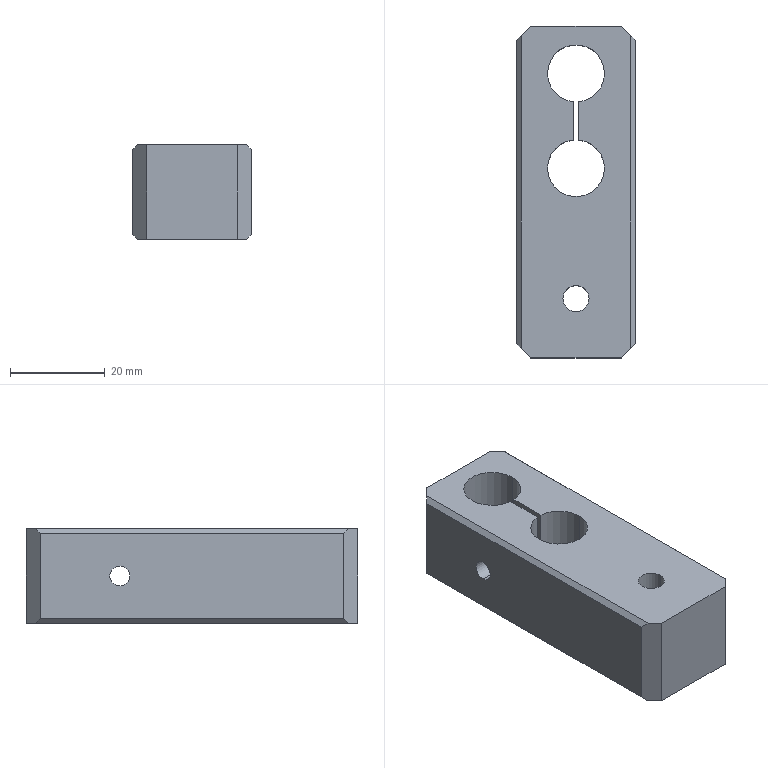Component | SolidWorks | 56-1 | 1 solid | 31 faces | box 25 x 70 x 20 mm | volume 28604 mm3 | plane 17 | cylinder 14 | commonest cylinder face diameters 12 x6 5.5 x4 4.2 x2 10 x2
build123d program:
from build123d import *

# Parameters (mm, degrees)
SKETCH1_W                                            = 25
SKETCH1_H                                            = 70
SKETCH1_R                                            = 6
BOSS_EXTRUDE1_DEPTH                                  = 20
CHAMFER1_SIZE                                        = 3
SKETCH2_W                                            = 1
SKETCH2_H                                            = 16.444
CUT_EXTRUDE1_DEPTH                                   = 20
M5_HEX_SOCKET_HEAD_CAP_SCREW_COUNTERBORE_D           = 5.5
M5_HEX_SOCKET_HEAD_CAP_SCREW_COUNTERBORE_DEPTH       = 12
M5_HEX_SOCKET_HEAD_CAP_SCREW_COUNTERBORE_CBORE_D     = 10
M5_HEX_SOCKET_HEAD_CAP_SCREW_COUNTERBORE_CBORE_DEPTH = 5.4
M5_TAPPED_HOLE1_D                                    = 4.2
M5_TAPPED_HOLE1_DEPTH                                = 14
M5_TAPPED_HOLE1_TIP                                  = 1.262
SKETCH6_R                                            = 2.75
CUT_EXTRUDE2_DEPTH                                   = 20
CHAMFER2_SIZE                                        = 3
CHAMFER3_SIZE                                        = 1


with BuildPart() as part:
    # Sketch1 → Boss-Extrude1 (new body)
    with BuildSketch(Plane.XY):
        with Locations((0, -5)):
            Rectangle(SKETCH1_W, SKETCH1_H)
        Circle(SKETCH1_R, mode=Mode.SUBTRACT)
        with Locations((0, 20)):
            Circle(SKETCH1_R, mode=Mode.SUBTRACT)
    extrude(amount=BOSS_EXTRUDE1_DEPTH)

    # Chamfer1
    chamfer1_edges = [part.edges().sort_by_distance(p)[0] for p in [
        (-12.5, 30, 10),
        (12.5, 30, 10),
    ]]
    chamfer(chamfer1_edges, length=CHAMFER1_SIZE)

    # Sketch2 → Cut-Extrude1 (cut)
    with BuildSketch(Plane.XY.offset(20)):
        with Locations((0, 8.896)):
            Rectangle(SKETCH2_W, SKETCH2_H)
    extrude(amount=-CUT_EXTRUDE1_DEPTH, mode=Mode.SUBTRACT)

    # M5 Hex Socket Head Cap Screw Counterbore
    with Locations(Plane(origin=(12.5, 10.226, 10), x_dir=(0, 1, 0), z_dir=(1, 0, 0))):
        with Locations((0, 0)):
            CounterBoreHole(M5_HEX_SOCKET_HEAD_CAP_SCREW_COUNTERBORE_D / 2, M5_HEX_SOCKET_HEAD_CAP_SCREW_COUNTERBORE_CBORE_D / 2, M5_HEX_SOCKET_HEAD_CAP_SCREW_COUNTERBORE_CBORE_DEPTH, depth=M5_HEX_SOCKET_HEAD_CAP_SCREW_COUNTERBORE_DEPTH)

    # M5 Tapped Hole1
    with Locations(Plane(origin=(-0.5, 0, 0), x_dir=(0, 0, -1), z_dir=(1, 0, 0))):
        with Locations((-10, 10.226)):
            Hole(M5_TAPPED_HOLE1_D / 2, depth=M5_TAPPED_HOLE1_DEPTH)
            with Locations((0, 0, -(M5_TAPPED_HOLE1_DEPTH + M5_TAPPED_HOLE1_TIP / 2))):  # 118° drill point
                Cone(0, M5_TAPPED_HOLE1_D / 2, M5_TAPPED_HOLE1_TIP, mode=Mode.SUBTRACT)

    # Sketch6 → Cut-Extrude2 (cut)
    with BuildSketch(Plane.XY.offset(20)):
        with Locations((0, -27.5)):
            Circle(SKETCH6_R)
    extrude(amount=-CUT_EXTRUDE2_DEPTH, mode=Mode.SUBTRACT)

    # Chamfer2
    chamfer2_edges = [part.edges().sort_by_distance(p)[0] for p in [
        (12.5, -40, 10),
        (-12.5, -40, 10),
    ]]
    chamfer(chamfer2_edges, length=CHAMFER2_SIZE)

    # Chamfer3
    chamfer3_edges = [part.edges().sort_by_distance(p)[0] for p in [
        (-12.5, -5, 0),
        (-12.5, -5, 20),
        (12.5, -5, 0),
        (12.5, -5, 20),
    ]]
    chamfer(chamfer3_edges, length=CHAMFER3_SIZE)


solid = part.part

# Placed as in the assembly
solid = solid.moved(Location((0, -38, 253.966), (0, 0, 0)))
STEP:
#1=COLOUR_RGB('',0.7922,0.8196,0.9333);
#2=FILL_AREA_STYLE_COLOUR('',#1);
#3=FILL_AREA_STYLE('',(#2));
#4=SURFACE_STYLE_FILL_AREA(#3);
#5=SURFACE_SIDE_STYLE('',(#4));
#6=SURFACE_STYLE_USAGE(.BOTH.,#5);
#7=PRESENTATION_STYLE_ASSIGNMENT((#6));
#8=CARTESIAN_POINT('',(-0.1083,-2.579,9.999));
#9=VERTEX_POINT('',#8);
#10=CARTESIAN_POINT('',(0.1083,-2.579,9.999));
#11=VERTEX_POINT('',#10);
#12=CARTESIAN_POINT('',(0.,-2.579,9.999));
#13=DIRECTION('',(0.,0.,1.));
#14=DIRECTION('',(1.,0.,0.));
#15=AXIS2_PLACEMENT_3D('',#12,#13,#14);
#16=CIRCLE('',#15,0.1083);
#17=EDGE_CURVE('',#9,#11,#16,.T.);
#18=ORIENTED_EDGE('',*,*,#17,.F.);
#19=CARTESIAN_POINT('',(-0.1083,-2.579,10.786));
#20=VERTEX_POINT('',#19);
#21=CARTESIAN_POINT('',(-0.1083,-2.579,9.999));
#22=DIRECTION('',(0.,0.,1.));
#23=VECTOR('',#22,39.37);
#24=LINE('',#21,#23);
#25=EDGE_CURVE('',#9,#20,#24,.T.);
#26=ORIENTED_EDGE('',*,*,#25,.T.);
#27=CARTESIAN_POINT('',(0.1083,-2.579,10.786));
#28=VERTEX_POINT('',#27);
#29=CARTESIAN_POINT('',(0.,-2.579,10.786));
#30=DIRECTION('',(0.,0.,1.));
#31=DIRECTION('',(1.,0.,0.));
#32=AXIS2_PLACEMENT_3D('',#29,#30,#31);
#33=CIRCLE('',#32,0.1083);
#34=EDGE_CURVE('',#20,#28,#33,.T.);
#35=ORIENTED_EDGE('',*,*,#34,.T.);
#36=CARTESIAN_POINT('',(0.1083,-2.579,9.999));
#37=DIRECTION('',(0.,0.,1.));
#38=VECTOR('',#37,39.37);
#39=LINE('',#36,#38);
#40=EDGE_CURVE('',#11,#28,#39,.T.);
#41=ORIENTED_EDGE('',*,*,#40,.F.);
#42=EDGE_LOOP('',(#18,#26,#35,#41));
#43=FACE_OUTER_BOUND('',#42,.T.);
#44=CARTESIAN_POINT('',(0.,-2.579,9.999));
#45=DIRECTION('',(0.,0.,1.));
#46=DIRECTION('',(1.,0.,0.));
#47=AXIS2_PLACEMENT_3D('',#44,#45,#46);
#48=CYLINDRICAL_SURFACE('',#47,0.1083);
#49=ADVANCED_FACE('',(#43),#48,.F.);
#50=CARTESIAN_POINT('',(-0.4921,-1.093,10.475));
#51=VERTEX_POINT('',#50);
#52=CARTESIAN_POINT('',(-0.4921,-1.093,10.31));
#53=VERTEX_POINT('',#52);
#54=CARTESIAN_POINT('',(-0.4921,-1.093,10.392));
#55=DIRECTION('',(1.,0.,0.));
#56=DIRECTION('',(0.,1.,0.));
#57=AXIS2_PLACEMENT_3D('',#54,#55,#56);
#58=CIRCLE('',#57,0.08268);
#59=EDGE_CURVE('',#51,#53,#58,.T.);
#60=ORIENTED_EDGE('',*,*,#59,.F.);
#61=CARTESIAN_POINT('',(-0.01969,-1.093,10.475));
#62=VERTEX_POINT('',#61);
#63=CARTESIAN_POINT('',(-0.01969,-1.093,10.475));
#64=DIRECTION('',(1.,0.,0.));
#65=VECTOR('',#64,39.37);
#66=LINE('',#63,#65);
#67=EDGE_CURVE('',#51,#62,#66,.T.);
#68=ORIENTED_EDGE('',*,*,#67,.T.);
#69=CARTESIAN_POINT('',(-0.01969,-1.093,10.31));
#70=VERTEX_POINT('',#69);
#71=CARTESIAN_POINT('',(-0.01969,-1.093,10.392));
#72=DIRECTION('',(1.,0.,0.));
#73=DIRECTION('',(0.,0.,-1.));
#74=AXIS2_PLACEMENT_3D('',#71,#72,#73);
#75=CIRCLE('',#74,0.08268);
#76=EDGE_CURVE('',#62,#70,#75,.T.);
#77=ORIENTED_EDGE('',*,*,#76,.T.);
#78=CARTESIAN_POINT('',(-0.01969,-1.093,10.31));
#79=DIRECTION('',(1.,0.,0.));
#80=VECTOR('',#79,39.37);
#81=LINE('',#78,#80);
#82=EDGE_CURVE('',#53,#70,#81,.T.);
#83=ORIENTED_EDGE('',*,*,#82,.F.);
#84=EDGE_LOOP('',(#60,#68,#77,#83));
#85=FACE_OUTER_BOUND('',#84,.T.);
#86=CARTESIAN_POINT('',(-0.01969,-1.093,10.392));
#87=DIRECTION('',(1.,0.,0.));
#88=DIRECTION('',(0.,0.,-1.));
#89=AXIS2_PLACEMENT_3D('',#86,#87,#88);
#90=CYLINDRICAL_SURFACE('',#89,0.08268);
#91=ADVANCED_FACE('',(#85),#90,.F.);
#92=CARTESIAN_POINT('',(0.2795,-1.093,10.589));
#93=VERTEX_POINT('',#92);
#94=CARTESIAN_POINT('',(0.2795,-1.093,10.196));
#95=VERTEX_POINT('',#94);
#96=CARTESIAN_POINT('',(0.2795,-1.093,10.392));
#97=DIRECTION('',(1.,0.,0.));
#98=DIRECTION('',(0.,0.,-1.));
#99=AXIS2_PLACEMENT_3D('',#96,#97,#98);
#100=CIRCLE('',#99,0.1969);
#101=EDGE_CURVE('',#93,#95,#100,.T.);
#102=ORIENTED_EDGE('',*,*,#101,.F.);
#103=CARTESIAN_POINT('',(0.4921,-1.093,10.589));
#104=VERTEX_POINT('',#103);
#105=CARTESIAN_POINT('',(0.4921,-1.093,10.589));
#106=DIRECTION('',(1.,0.,0.));
#107=VECTOR('',#106,39.37);
#108=LINE('',#105,#107);
#109=EDGE_CURVE('',#93,#104,#108,.T.);
#110=ORIENTED_EDGE('',*,*,#109,.T.);
#111=CARTESIAN_POINT('',(0.4921,-1.093,10.196));
#112=VERTEX_POINT('',#111);
#113=CARTESIAN_POINT('',(0.4921,-1.093,10.392));
#114=DIRECTION('',(1.,0.,0.));
#115=DIRECTION('',(0.,0.,-1.));
#116=AXIS2_PLACEMENT_3D('',#113,#114,#115);
#117=CIRCLE('',#116,0.1969);
#118=EDGE_CURVE('',#104,#112,#117,.T.);
#119=ORIENTED_EDGE('',*,*,#118,.T.);
#120=CARTESIAN_POINT('',(0.4921,-1.093,10.196));
#121=DIRECTION('',(1.,0.,0.));
#122=VECTOR('',#121,39.37);
#123=LINE('',#120,#122);
#124=EDGE_CURVE('',#95,#112,#123,.T.);
#125=ORIENTED_EDGE('',*,*,#124,.F.);
#126=EDGE_LOOP('',(#102,#110,#119,#125));
#127=FACE_OUTER_BOUND('',#126,.T.);
#128=CARTESIAN_POINT('',(0.4921,-1.093,10.392));
#129=DIRECTION('',(1.,0.,0.));
#130=DIRECTION('',(0.,0.,-1.));
#131=AXIS2_PLACEMENT_3D('',#128,#129,#130);
#132=CYLINDRICAL_SURFACE('',#131,0.1969);
#133=ADVANCED_FACE('',(#127),#132,.F.);
#134=CARTESIAN_POINT('',(0.01969,-1.093,10.501));
#135=VERTEX_POINT('',#134);
#136=CARTESIAN_POINT('',(0.01969,-1.093,10.284));
#137=VERTEX_POINT('',#136);
#138=CARTESIAN_POINT('',(0.01969,-1.093,10.392));
#139=DIRECTION('',(1.,0.,0.));
#140=DIRECTION('',(-0.,1.,0.));
#141=AXIS2_PLACEMENT_3D('',#138,#139,#140);
#142=CIRCLE('',#141,0.1083);
#143=EDGE_CURVE('',#135,#137,#142,.T.);
#144=ORIENTED_EDGE('',*,*,#143,.F.);
#145=CARTESIAN_POINT('',(0.2795,-1.093,10.501));
#146=VERTEX_POINT('',#145);
#147=CARTESIAN_POINT('',(0.4921,-1.093,10.501));
#148=DIRECTION('',(1.,0.,0.));
#149=VECTOR('',#148,39.37);
#150=LINE('',#147,#149);
#151=EDGE_CURVE('',#135,#146,#150,.T.);
#152=ORIENTED_EDGE('',*,*,#151,.T.);
#153=CARTESIAN_POINT('',(0.2795,-1.093,10.284));
#154=VERTEX_POINT('',#153);
#155=CARTESIAN_POINT('',(0.2795,-1.093,10.392));
#156=DIRECTION('',(1.,0.,0.));
#157=DIRECTION('',(0.,0.,-1.));
#158=AXIS2_PLACEMENT_3D('',#155,#156,#157);
#159=CIRCLE('',#158,0.1083);
#160=EDGE_CURVE('',#146,#154,#159,.T.);
#161=ORIENTED_EDGE('',*,*,#160,.T.);
#162=CARTESIAN_POINT('',(0.4921,-1.093,10.284));
#163=DIRECTION('',(1.,0.,0.));
#164=VECTOR('',#163,39.37);
#165=LINE('',#162,#164);
#166=EDGE_CURVE('',#137,#154,#165,.T.);
#167=ORIENTED_EDGE('',*,*,#166,.F.);
#168=EDGE_LOOP('',(#144,#152,#161,#167));
#169=FACE_OUTER_BOUND('',#168,.T.);
#170=CARTESIAN_POINT('',(0.4921,-1.093,10.392));
#171=DIRECTION('',(1.,0.,0.));
#172=DIRECTION('',(0.,0.,-1.));
#173=AXIS2_PLACEMENT_3D('',#170,#171,#172);
#174=CYLINDRICAL_SURFACE('',#173,0.1083);
#175=ADVANCED_FACE('',(#169),#174,.F.);
#176=CARTESIAN_POINT('',(0.01969,-0.9441,10.786));
#177=VERTEX_POINT('',#176);
#178=CARTESIAN_POINT('',(0.2362,-0.7087,10.786));
#179=VERTEX_POINT('',#178);
#180=CARTESIAN_POINT('',(-0.,-0.7087,10.786));
#181=DIRECTION('',(0.,0.,1.));
#182=DIRECTION('',(1.,0.,0.));
#183=AXIS2_PLACEMENT_3D('',#180,#181,#182);
#184=CIRCLE('',#183,0.2362);
#185=EDGE_CURVE('',#177,#179,#184,.T.);
#186=ORIENTED_EDGE('',*,*,#185,.T.);
#187=CARTESIAN_POINT('',(0.2362,-0.7087,9.999));
#188=VERTEX_POINT('',#187);
#189=CARTESIAN_POINT('',(0.2362,-0.7087,10.786));
#190=DIRECTION('',(0.,0.,-1.));
#191=VECTOR('',#190,39.37);
#192=LINE('',#189,#191);
#193=EDGE_CURVE('',#179,#188,#192,.T.);
#194=ORIENTED_EDGE('',*,*,#193,.T.);
#195=CARTESIAN_POINT('',(0.01969,-0.9441,9.999));
#196=VERTEX_POINT('',#195);
#197=CARTESIAN_POINT('',(-0.,-0.7087,9.999));
#198=DIRECTION('',(0.,0.,1.));
#199=DIRECTION('',(1.,0.,0.));
#200=AXIS2_PLACEMENT_3D('',#197,#198,#199);
#201=CIRCLE('',#200,0.2362);
#202=EDGE_CURVE('',#196,#188,#201,.T.);
#203=ORIENTED_EDGE('',*,*,#202,.F.);
#204=CARTESIAN_POINT('',(0.01969,-0.9441,10.786));
#205=DIRECTION('',(0.,0.,-1.));
#206=VECTOR('',#205,39.37);
#207=LINE('',#204,#206);
#208=EDGE_CURVE('',#177,#196,#207,.T.);
#209=ORIENTED_EDGE('',*,*,#208,.F.);
#210=EDGE_LOOP('',(#186,#194,#203,#209));
#211=FACE_OUTER_BOUND('',#210,.T.);
#212=CARTESIAN_POINT('',(-0.,-0.7087,10.786));
#213=DIRECTION('',(0.,0.,-1.));
#214=DIRECTION('',(-1.,0.,0.));
#215=AXIS2_PLACEMENT_3D('',#212,#213,#214);
#216=CYLINDRICAL_SURFACE('',#215,0.2362);
#217=ADVANCED_FACE('',(#211),#216,.F.);
#218=ORIENTED_EDGE('',*,*,#193,.F.);
#219=CARTESIAN_POINT('',(-0.2362,-0.7087,10.786));
#220=VERTEX_POINT('',#219);
#221=CARTESIAN_POINT('',(-0.,-0.7087,10.786));
#222=DIRECTION('',(0.,0.,1.));
#223=DIRECTION('',(1.,0.,0.));
#224=AXIS2_PLACEMENT_3D('',#221,#222,#223);
#225=CIRCLE('',#224,0.2362);
#226=EDGE_CURVE('',#179,#220,#225,.T.);
#227=ORIENTED_EDGE('',*,*,#226,.T.);
#228=CARTESIAN_POINT('',(-0.2362,-0.7087,9.999));
#229=VERTEX_POINT('',#228);
#230=CARTESIAN_POINT('',(-0.2362,-0.7087,10.786));
#231=DIRECTION('',(0.,0.,-1.));
#232=VECTOR('',#231,39.37);
#233=LINE('',#230,#232);
#234=EDGE_CURVE('',#220,#229,#233,.T.);
#235=ORIENTED_EDGE('',*,*,#234,.T.);
#236=CARTESIAN_POINT('',(-0.,-0.7087,9.999));
#237=DIRECTION('',(0.,0.,1.));
#238=DIRECTION('',(1.,0.,0.));
#239=AXIS2_PLACEMENT_3D('',#236,#237,#238);
#240=CIRCLE('',#239,0.2362);
#241=EDGE_CURVE('',#188,#229,#240,.T.);
#242=ORIENTED_EDGE('',*,*,#241,.F.);
#243=EDGE_LOOP('',(#218,#227,#235,#242));
#244=FACE_OUTER_BOUND('',#243,.T.);
#245=CARTESIAN_POINT('',(-0.,-0.7087,10.786));
#246=DIRECTION('',(0.,0.,-1.));
#247=DIRECTION('',(-1.,0.,0.));
#248=AXIS2_PLACEMENT_3D('',#245,#246,#247);
#249=CYLINDRICAL_SURFACE('',#248,0.2362);
#250=ADVANCED_FACE('',(#244),#249,.F.);
#251=CARTESIAN_POINT('',(-0.2362,-1.496,10.786));
#252=VERTEX_POINT('',#251);
#253=CARTESIAN_POINT('',(0.2362,-1.496,10.786));
#254=VERTEX_POINT('',#253);
#255=CARTESIAN_POINT('',(0.,-1.496,10.786));
#256=DIRECTION('',(0.,0.,1.));
#257=DIRECTION('',(1.,0.,0.));
#258=AXIS2_PLACEMENT_3D('',#255,#256,#257);
#259=CIRCLE('',#258,0.2362);
#260=EDGE_CURVE('',#252,#254,#259,.T.);
#261=ORIENTED_EDGE('',*,*,#260,.T.);
#262=CARTESIAN_POINT('',(0.2362,-1.496,9.999));
#263=VERTEX_POINT('',#262);
#264=CARTESIAN_POINT('',(0.2362,-1.496,10.786));
#265=DIRECTION('',(0.,0.,-1.));
#266=VECTOR('',#265,39.37);
#267=LINE('',#264,#266);
#268=EDGE_CURVE('',#254,#263,#267,.T.);
#269=ORIENTED_EDGE('',*,*,#268,.T.);
#270=CARTESIAN_POINT('',(-0.2362,-1.496,9.999));
#271=VERTEX_POINT('',#270);
#272=CARTESIAN_POINT('',(0.,-1.496,9.999));
#273=DIRECTION('',(0.,0.,1.));
#274=DIRECTION('',(1.,0.,0.));
#275=AXIS2_PLACEMENT_3D('',#272,#273,#274);
#276=CIRCLE('',#275,0.2362);
#277=EDGE_CURVE('',#271,#263,#276,.T.);
#278=ORIENTED_EDGE('',*,*,#277,.F.);
#279=CARTESIAN_POINT('',(-0.2362,-1.496,10.786));
#280=DIRECTION('',(0.,0.,-1.));
#281=VECTOR('',#280,39.37);
#282=LINE('',#279,#281);
#283=EDGE_CURVE('',#252,#271,#282,.T.);
#284=ORIENTED_EDGE('',*,*,#283,.F.);
#285=EDGE_LOOP('',(#261,#269,#278,#284));
#286=FACE_OUTER_BOUND('',#285,.T.);
#287=CARTESIAN_POINT('',(0.,-1.496,10.786));
#288=DIRECTION('',(0.,0.,-1.));
#289=DIRECTION('',(-1.,0.,0.));
#290=AXIS2_PLACEMENT_3D('',#287,#288,#289);
#291=CYLINDRICAL_SURFACE('',#290,0.2362);
#292=ADVANCED_FACE('',(#286),#291,.F.);
#293=CARTESIAN_POINT('',(-0.01969,-1.261,10.786));
#294=VERTEX_POINT('',#293);
#295=CARTESIAN_POINT('',(0.,-1.496,10.786));
#296=DIRECTION('',(0.,0.,1.));
#297=DIRECTION('',(1.,0.,0.));
#298=AXIS2_PLACEMENT_3D('',#295,#296,#297);
#299=CIRCLE('',#298,0.2362);
#300=EDGE_CURVE('',#294,#252,#299,.T.);
#301=ORIENTED_EDGE('',*,*,#300,.T.);
#302=ORIENTED_EDGE('',*,*,#283,.T.);
#303=CARTESIAN_POINT('',(-0.01969,-1.261,9.999));
#304=VERTEX_POINT('',#303);
#305=CARTESIAN_POINT('',(0.,-1.496,9.999));
#306=DIRECTION('',(0.,0.,1.));
#307=DIRECTION('',(1.,0.,0.));
#308=AXIS2_PLACEMENT_3D('',#305,#306,#307);
#309=CIRCLE('',#308,0.2362);
#310=EDGE_CURVE('',#304,#271,#309,.T.);
#311=ORIENTED_EDGE('',*,*,#310,.F.);
#312=CARTESIAN_POINT('',(-0.01969,-1.261,10.786));
#313=DIRECTION('',(0.,0.,-1.));
#314=VECTOR('',#313,39.37);
#315=LINE('',#312,#314);
#316=EDGE_CURVE('',#294,#304,#315,.T.);
#317=ORIENTED_EDGE('',*,*,#316,.F.);
#318=EDGE_LOOP('',(#301,#302,#311,#317));
#319=FACE_OUTER_BOUND('',#318,.T.);
#320=CARTESIAN_POINT('',(0.,-1.496,10.786));
#321=DIRECTION('',(0.,0.,-1.));
#322=DIRECTION('',(-1.,0.,0.));
#323=AXIS2_PLACEMENT_3D('',#320,#321,#322);
#324=CYLINDRICAL_SURFACE('',#323,0.2362);
#325=ADVANCED_FACE('',(#319),#324,.F.);
#326=CARTESIAN_POINT('',(0.4921,-2.953,10.747));
#327=VERTEX_POINT('',#326);
#328=CARTESIAN_POINT('',(0.4921,-2.953,10.038));
#329=VERTEX_POINT('',#328);
#330=CARTESIAN_POINT('',(0.4921,-2.953,10.786));
#331=DIRECTION('',(0.,0.,-1.));
#332=VECTOR('',#331,39.37);
#333=LINE('',#330,#332);
#334=EDGE_CURVE('',#327,#329,#333,.T.);
#335=ORIENTED_EDGE('',*,*,#334,.T.);
#336=CARTESIAN_POINT('',(0.4921,-0.4331,10.038));
#337=VERTEX_POINT('',#336);
#338=CARTESIAN_POINT('',(0.4921,-0.315,10.038));
#339=DIRECTION('',(-0.,1.,0.));
#340=VECTOR('',#339,39.37);
#341=LINE('',#338,#340);
#342=EDGE_CURVE('',#329,#337,#341,.T.);
#343=ORIENTED_EDGE('',*,*,#342,.T.);
#344=CARTESIAN_POINT('',(0.4921,-0.4331,10.747));
#345=VERTEX_POINT('',#344);
#346=CARTESIAN_POINT('',(0.4921,-0.4331,10.786));
#347=DIRECTION('',(0.,0.,1.));
#348=VECTOR('',#347,39.37);
#349=LINE('',#346,#348);
#350=EDGE_CURVE('',#337,#345,#349,.T.);
#351=ORIENTED_EDGE('',*,*,#350,.T.);
#352=CARTESIAN_POINT('',(0.4921,-2.953,10.747));
#353=DIRECTION('',(0.,-1.,0.));
#354=VECTOR('',#353,39.37);
#355=LINE('',#352,#354);
#356=EDGE_CURVE('',#345,#327,#355,.T.);
#357=ORIENTED_EDGE('',*,*,#356,.T.);
#358=EDGE_LOOP('',(#335,#343,#351,#357));
#359=FACE_OUTER_BOUND('',#358,.T.);
#360=CARTESIAN_POINT('',(0.4921,-1.093,10.392));
#361=DIRECTION('',(1.,0.,0.));
#362=DIRECTION('',(0.,0.,-1.));
#363=AXIS2_PLACEMENT_3D('',#360,#361,#362);
#364=CIRCLE('',#363,0.1969);
#365=EDGE_CURVE('',#112,#104,#364,.T.);
#366=ORIENTED_EDGE('',*,*,#365,.F.);
#367=ORIENTED_EDGE('',*,*,#118,.F.);
#368=EDGE_LOOP('',(#366,#367));
#369=FACE_BOUND('',#368,.T.);
#370=CARTESIAN_POINT('',(0.4921,-0.315,10.786));
#371=DIRECTION('',(-1.,-0.,0.));
#372=DIRECTION('',(0.,-1.,0.));
#373=AXIS2_PLACEMENT_3D('',#370,#371,#372);
#374=PLANE('',#373);
#375=ADVANCED_FACE('',(#359,#369),#374,.F.);
#376=CARTESIAN_POINT('',(0.,-2.579,10.786));
#377=DIRECTION('',(0.,0.,1.));
#378=DIRECTION('',(1.,0.,0.));
#379=AXIS2_PLACEMENT_3D('',#376,#377,#378);
#380=CIRCLE('',#379,0.1083);
#381=EDGE_CURVE('',#28,#20,#380,.T.);
#382=ORIENTED_EDGE('',*,*,#381,.F.);
#383=ORIENTED_EDGE('',*,*,#34,.F.);
#384=EDGE_LOOP('',(#382,#383));
#385=FACE_BOUND('',#384,.T.);
#386=CARTESIAN_POINT('',(-0.01969,-0.9441,10.786));
#387=VERTEX_POINT('',#386);
#388=CARTESIAN_POINT('',(-0.01969,-0.8221,10.786));
#389=DIRECTION('',(0.,-1.,0.));
#390=VECTOR('',#389,39.37);
#391=LINE('',#388,#390);
#392=EDGE_CURVE('',#387,#294,#391,.T.);
#393=ORIENTED_EDGE('',*,*,#392,.F.);
#394=CARTESIAN_POINT('',(-0.,-0.7087,10.786));
#395=DIRECTION('',(0.,0.,1.));
#396=DIRECTION('',(1.,0.,0.));
#397=AXIS2_PLACEMENT_3D('',#394,#395,#396);
#398=CIRCLE('',#397,0.2362);
#399=EDGE_CURVE('',#220,#387,#398,.T.);
#400=ORIENTED_EDGE('',*,*,#399,.F.);
#401=ORIENTED_EDGE('',*,*,#226,.F.);
#402=ORIENTED_EDGE('',*,*,#185,.F.);
#403=CARTESIAN_POINT('',(0.01969,-1.261,10.786));
#404=VERTEX_POINT('',#403);
#405=CARTESIAN_POINT('',(0.01969,-0.8221,10.786));
#406=DIRECTION('',(-0.,1.,0.));
#407=VECTOR('',#406,39.37);
#408=LINE('',#405,#407);
#409=EDGE_CURVE('',#404,#177,#408,.T.);
#410=ORIENTED_EDGE('',*,*,#409,.F.);
#411=CARTESIAN_POINT('',(0.,-1.496,10.786));
#412=DIRECTION('',(0.,0.,1.));
#413=DIRECTION('',(1.,0.,0.));
#414=AXIS2_PLACEMENT_3D('',#411,#412,#413);
#415=CIRCLE('',#414,0.2362);
#416=EDGE_CURVE('',#254,#404,#415,.T.);
#417=ORIENTED_EDGE('',*,*,#416,.F.);
#418=ORIENTED_EDGE('',*,*,#260,.F.);
#419=ORIENTED_EDGE('',*,*,#300,.F.);
#420=EDGE_LOOP('',(#393,#400,#401,#402,#410,#417,#418,#419));
#421=FACE_BOUND('',#420,.T.);
#422=CARTESIAN_POINT('',(-0.374,-0.315,10.786));
#423=VERTEX_POINT('',#422);
#424=CARTESIAN_POINT('',(-0.4528,-0.3937,10.786));
#425=VERTEX_POINT('',#424);
#426=CARTESIAN_POINT('',(-0.7776,-0.7185,10.786));
#427=DIRECTION('',(-0.7071,-0.7071,0.));
#428=VECTOR('',#427,39.37);
#429=LINE('',#426,#428);
#430=EDGE_CURVE('',#423,#425,#429,.T.);
#431=ORIENTED_EDGE('',*,*,#430,.T.);
#432=CARTESIAN_POINT('',(-0.4528,-2.992,10.786));
#433=VERTEX_POINT('',#432);
#434=CARTESIAN_POINT('',(-0.4528,-2.953,10.786));
#435=DIRECTION('',(0.,-1.,0.));
#436=VECTOR('',#435,39.37);
#437=LINE('',#434,#436);
#438=EDGE_CURVE('',#425,#433,#437,.T.);
#439=ORIENTED_EDGE('',*,*,#438,.T.);
#440=CARTESIAN_POINT('',(-0.374,-3.071,10.786));
#441=VERTEX_POINT('',#440);
#442=CARTESIAN_POINT('',(-0.9744,-2.47,10.786));
#443=DIRECTION('',(0.7071,-0.7071,0.));
#444=VECTOR('',#443,39.37);
#445=LINE('',#442,#444);
#446=EDGE_CURVE('',#433,#441,#445,.T.);
#447=ORIENTED_EDGE('',*,*,#446,.T.);
#448=CARTESIAN_POINT('',(0.374,-3.071,10.786));
#449=VERTEX_POINT('',#448);
#450=CARTESIAN_POINT('',(-0.4921,-3.071,10.786));
#451=DIRECTION('',(1.,-0.,0.));
#452=VECTOR('',#451,39.37);
#453=LINE('',#450,#452);
#454=EDGE_CURVE('',#441,#449,#453,.T.);
#455=ORIENTED_EDGE('',*,*,#454,.T.);
#456=CARTESIAN_POINT('',(0.4528,-2.992,10.786));
#457=VERTEX_POINT('',#456);
#458=CARTESIAN_POINT('',(0.9744,-2.47,10.786));
#459=DIRECTION('',(0.7071,0.7071,0.));
#460=VECTOR('',#459,39.37);
#461=LINE('',#458,#460);
#462=EDGE_CURVE('',#449,#457,#461,.T.);
#463=ORIENTED_EDGE('',*,*,#462,.T.);
#464=CARTESIAN_POINT('',(0.4528,-0.3937,10.786));
#465=VERTEX_POINT('',#464);
#466=CARTESIAN_POINT('',(0.4528,-0.4331,10.786));
#467=DIRECTION('',(-0.,1.,0.));
#468=VECTOR('',#467,39.37);
#469=LINE('',#466,#468);
#470=EDGE_CURVE('',#457,#465,#469,.T.);
#471=ORIENTED_EDGE('',*,*,#470,.T.);
#472=CARTESIAN_POINT('',(0.374,-0.315,10.786));
#473=VERTEX_POINT('',#472);
#474=CARTESIAN_POINT('',(0.7776,-0.7185,10.786));
#475=DIRECTION('',(-0.7071,0.7071,0.));
#476=VECTOR('',#475,39.37);
#477=LINE('',#474,#476);
#478=EDGE_CURVE('',#465,#473,#477,.T.);
#479=ORIENTED_EDGE('',*,*,#478,.T.);
#480=CARTESIAN_POINT('',(-0.4921,-0.315,10.786));
#481=DIRECTION('',(-1.,0.,0.));
#482=VECTOR('',#481,39.37);
#483=LINE('',#480,#482);
#484=EDGE_CURVE('',#473,#423,#483,.T.);
#485=ORIENTED_EDGE('',*,*,#484,.T.);
#486=EDGE_LOOP('',(#431,#439,#447,#455,#463,#471,#479,#485));
#487=FACE_OUTER_BOUND('',#486,.T.);
#488=CARTESIAN_POINT('',(0.,-1.496,10.786));
#489=DIRECTION('',(0.,0.,1.));
#490=DIRECTION('',(1.,0.,0.));
#491=AXIS2_PLACEMENT_3D('',#488,#489,#490);
#492=PLANE('',#491);
#493=ADVANCED_FACE('',(#385,#421,#487),#492,.T.);
#494=CARTESIAN_POINT('',(0.,-2.579,9.999));
#495=DIRECTION('',(0.,0.,1.));
#496=DIRECTION('',(1.,0.,0.));
#497=AXIS2_PLACEMENT_3D('',#494,#495,#496);
#498=CIRCLE('',#497,0.1083);
#499=EDGE_CURVE('',#11,#9,#498,.T.);
#500=ORIENTED_EDGE('',*,*,#499,.T.);
#501=ORIENTED_EDGE('',*,*,#17,.T.);
#502=EDGE_LOOP('',(#500,#501));
#503=FACE_BOUND('',#502,.T.);
#504=CARTESIAN_POINT('',(-0.374,-3.071,9.999));
#505=VERTEX_POINT('',#504);
#506=CARTESIAN_POINT('',(-0.4528,-2.992,9.999));
#507=VERTEX_POINT('',#506);
#508=CARTESIAN_POINT('',(-0.374,-3.071,9.999));
#509=DIRECTION('',(-0.7071,0.7071,0.));
#510=VECTOR('',#509,39.37);
#511=LINE('',#508,#510);
#512=EDGE_CURVE('',#505,#507,#511,.T.);
#513=ORIENTED_EDGE('',*,*,#512,.T.);
#514=CARTESIAN_POINT('',(-0.4528,-0.3937,9.999));
#515=VERTEX_POINT('',#514);
#516=CARTESIAN_POINT('',(-0.4528,-1.496,9.999));
#517=DIRECTION('',(-0.,1.,0.));
#518=VECTOR('',#517,39.37);
#519=LINE('',#516,#518);
#520=EDGE_CURVE('',#507,#515,#519,.T.);
#521=ORIENTED_EDGE('',*,*,#520,.T.);
#522=CARTESIAN_POINT('',(-0.374,-0.315,9.999));
#523=VERTEX_POINT('',#522);
#524=CARTESIAN_POINT('',(-0.4921,-0.4331,9.999));
#525=DIRECTION('',(0.7071,0.7071,0.));
#526=VECTOR('',#525,39.37);
#527=LINE('',#524,#526);
#528=EDGE_CURVE('',#515,#523,#527,.T.);
#529=ORIENTED_EDGE('',*,*,#528,.T.);
#530=CARTESIAN_POINT('',(0.374,-0.315,9.999));
#531=VERTEX_POINT('',#530);
#532=CARTESIAN_POINT('',(-0.4921,-0.315,9.999));
#533=DIRECTION('',(-1.,0.,0.));
#534=VECTOR('',#533,39.37);
#535=LINE('',#532,#534);
#536=EDGE_CURVE('',#531,#523,#535,.T.);
#537=ORIENTED_EDGE('',*,*,#536,.F.);
#538=CARTESIAN_POINT('',(0.4528,-0.3937,9.999));
#539=VERTEX_POINT('',#538);
#540=CARTESIAN_POINT('',(0.374,-0.315,9.999));
#541=DIRECTION('',(0.7071,-0.7071,0.));
#542=VECTOR('',#541,39.37);
#543=LINE('',#540,#542);
#544=EDGE_CURVE('',#531,#539,#543,.T.);
#545=ORIENTED_EDGE('',*,*,#544,.T.);
#546=CARTESIAN_POINT('',(0.4528,-2.992,9.999));
#547=VERTEX_POINT('',#546);
#548=CARTESIAN_POINT('',(0.4528,-1.496,9.999));
#549=DIRECTION('',(0.,-1.,0.));
#550=VECTOR('',#549,39.37);
#551=LINE('',#548,#550);
#552=EDGE_CURVE('',#539,#547,#551,.T.);
#553=ORIENTED_EDGE('',*,*,#552,.T.);
#554=CARTESIAN_POINT('',(0.374,-3.071,9.999));
#555=VERTEX_POINT('',#554);
#556=CARTESIAN_POINT('',(0.4921,-2.953,9.999));
#557=DIRECTION('',(-0.7071,-0.7071,0.));
#558=VECTOR('',#557,39.37);
#559=LINE('',#556,#558);
#560=EDGE_CURVE('',#547,#555,#559,.T.);
#561=ORIENTED_EDGE('',*,*,#560,.T.);
#562=CARTESIAN_POINT('',(-0.4921,-3.071,9.999));
#563=DIRECTION('',(1.,-0.,0.));
#564=VECTOR('',#563,39.37);
#565=LINE('',#562,#564);
#566=EDGE_CURVE('',#505,#555,#565,.T.);
#567=ORIENTED_EDGE('',*,*,#566,.F.);
#568=EDGE_LOOP('',(#513,#521,#529,#537,#545,#553,#561,#567));
#569=FACE_OUTER_BOUND('',#568,.T.);
#570=ORIENTED_EDGE('',*,*,#202,.T.);
#571=ORIENTED_EDGE('',*,*,#241,.T.);
#572=CARTESIAN_POINT('',(-0.01969,-0.9441,9.999));
#573=VERTEX_POINT('',#572);
#574=CARTESIAN_POINT('',(-0.,-0.7087,9.999));
#575=DIRECTION('',(0.,0.,1.));
#576=DIRECTION('',(1.,0.,0.));
#577=AXIS2_PLACEMENT_3D('',#574,#575,#576);
#578=CIRCLE('',#577,0.2362);
#579=EDGE_CURVE('',#229,#573,#578,.T.);
#580=ORIENTED_EDGE('',*,*,#579,.T.);
#581=CARTESIAN_POINT('',(-0.01969,-0.8221,9.999));
#582=DIRECTION('',(0.,-1.,0.));
#583=VECTOR('',#582,39.37);
#584=LINE('',#581,#583);
#585=EDGE_CURVE('',#573,#304,#584,.T.);
#586=ORIENTED_EDGE('',*,*,#585,.T.);
#587=ORIENTED_EDGE('',*,*,#310,.T.);
#588=ORIENTED_EDGE('',*,*,#277,.T.);
#589=CARTESIAN_POINT('',(0.01969,-1.261,9.999));
#590=VERTEX_POINT('',#589);
#591=CARTESIAN_POINT('',(0.,-1.496,9.999));
#592=DIRECTION('',(0.,0.,1.));
#593=DIRECTION('',(1.,0.,0.));
#594=AXIS2_PLACEMENT_3D('',#591,#592,#593);
#595=CIRCLE('',#594,0.2362);
#596=EDGE_CURVE('',#263,#590,#595,.T.);
#597=ORIENTED_EDGE('',*,*,#596,.T.);
#598=CARTESIAN_POINT('',(0.01969,-0.8221,9.999));
#599=DIRECTION('',(-0.,1.,0.));
#600=VECTOR('',#599,39.37);
#601=LINE('',#598,#600);
#602=EDGE_CURVE('',#590,#196,#601,.T.);
#603=ORIENTED_EDGE('',*,*,#602,.T.);
#604=EDGE_LOOP('',(#570,#571,#580,#586,#587,#588,#597,#603));
#605=FACE_BOUND('',#604,.T.);
#606=CARTESIAN_POINT('',(0.,-1.496,9.999));
#607=DIRECTION('',(0.,0.,1.));
#608=DIRECTION('',(1.,0.,0.));
#609=AXIS2_PLACEMENT_3D('',#606,#607,#608);
#610=PLANE('',#609);
#611=ADVANCED_FACE('',(#503,#569,#605),#610,.F.);
#612=CARTESIAN_POINT('',(-0.4921,-1.093,10.392));
#613=DIRECTION('',(1.,0.,0.));
#614=DIRECTION('',(0.,1.,0.));
#615=AXIS2_PLACEMENT_3D('',#612,#613,#614);
#616=CIRCLE('',#615,0.08268);
#617=EDGE_CURVE('',#53,#51,#616,.T.);
#618=ORIENTED_EDGE('',*,*,#617,.T.);
#619=ORIENTED_EDGE('',*,*,#59,.T.);
#620=EDGE_LOOP('',(#618,#619));
#621=FACE_BOUND('',#620,.T.);
#622=CARTESIAN_POINT('',(-0.4921,-0.4331,10.747));
#623=VERTEX_POINT('',#622);
#624=CARTESIAN_POINT('',(-0.4921,-0.4331,10.038));
#625=VERTEX_POINT('',#624);
#626=CARTESIAN_POINT('',(-0.4921,-0.4331,10.786));
#627=DIRECTION('',(0.,0.,-1.));
#628=VECTOR('',#627,39.37);
#629=LINE('',#626,#628);
#630=EDGE_CURVE('',#623,#625,#629,.T.);
#631=ORIENTED_EDGE('',*,*,#630,.T.);
#632=CARTESIAN_POINT('',(-0.4921,-2.953,10.038));
#633=VERTEX_POINT('',#632);
#634=CARTESIAN_POINT('',(-0.4921,-0.315,10.038));
#635=DIRECTION('',(0.,-1.,0.));
#636=VECTOR('',#635,39.37);
#637=LINE('',#634,#636);
#638=EDGE_CURVE('',#625,#633,#637,.T.);
#639=ORIENTED_EDGE('',*,*,#638,.T.);
#640=CARTESIAN_POINT('',(-0.4921,-2.953,10.747));
#641=VERTEX_POINT('',#640);
#642=CARTESIAN_POINT('',(-0.4921,-2.953,10.786));
#643=DIRECTION('',(0.,0.,1.));
#644=VECTOR('',#643,39.37);
#645=LINE('',#642,#644);
#646=EDGE_CURVE('',#633,#641,#645,.T.);
#647=ORIENTED_EDGE('',*,*,#646,.T.);
#648=CARTESIAN_POINT('',(-0.4921,-0.4331,10.747));
#649=DIRECTION('',(-0.,1.,0.));
#650=VECTOR('',#649,39.37);
#651=LINE('',#648,#650);
#652=EDGE_CURVE('',#641,#623,#651,.T.);
#653=ORIENTED_EDGE('',*,*,#652,.T.);
#654=EDGE_LOOP('',(#631,#639,#647,#653));
#655=FACE_OUTER_BOUND('',#654,.T.);
#656=CARTESIAN_POINT('',(-0.4921,-0.315,10.786));
#657=DIRECTION('',(1.,0.,0.));
#658=DIRECTION('',(-0.,1.,0.));
#659=AXIS2_PLACEMENT_3D('',#656,#657,#658);
#660=PLANE('',#659);
#661=ADVANCED_FACE('',(#621,#655),#660,.F.);
#662=ORIENTED_EDGE('',*,*,#566,.T.);
#663=CARTESIAN_POINT('',(0.374,-3.071,10.786));
#664=DIRECTION('',(0.,0.,1.));
#665=VECTOR('',#664,39.37);
#666=LINE('',#663,#665);
#667=EDGE_CURVE('',#555,#449,#666,.T.);
#668=ORIENTED_EDGE('',*,*,#667,.T.);
#669=ORIENTED_EDGE('',*,*,#454,.F.);
#670=CARTESIAN_POINT('',(-0.374,-3.071,10.786));
#671=DIRECTION('',(0.,0.,-1.));
#672=VECTOR('',#671,39.37);
#673=LINE('',#670,#672);
#674=EDGE_CURVE('',#441,#505,#673,.T.);
#675=ORIENTED_EDGE('',*,*,#674,.T.);
#676=EDGE_LOOP('',(#662,#668,#669,#675));
#677=FACE_OUTER_BOUND('',#676,.T.);
#678=CARTESIAN_POINT('',(-0.4921,-3.071,10.786));
#679=DIRECTION('',(0.,1.,0.));
#680=DIRECTION('',(-1.,0.,0.));
#681=AXIS2_PLACEMENT_3D('',#678,#679,#680);
#682=PLANE('',#681);
#683=ADVANCED_FACE('',(#677),#682,.F.);
#684=ORIENTED_EDGE('',*,*,#536,.T.);
#685=CARTESIAN_POINT('',(-0.374,-0.315,10.786));
#686=DIRECTION('',(0.,0.,1.));
#687=VECTOR('',#686,39.37);
#688=LINE('',#685,#687);
#689=EDGE_CURVE('',#523,#423,#688,.T.);
#690=ORIENTED_EDGE('',*,*,#689,.T.);
#691=ORIENTED_EDGE('',*,*,#484,.F.);
#692=CARTESIAN_POINT('',(0.374,-0.315,10.786));
#693=DIRECTION('',(0.,0.,-1.));
#694=VECTOR('',#693,39.37);
#695=LINE('',#692,#694);
#696=EDGE_CURVE('',#473,#531,#695,.T.);
#697=ORIENTED_EDGE('',*,*,#696,.T.);
#698=EDGE_LOOP('',(#684,#690,#691,#697));
#699=FACE_OUTER_BOUND('',#698,.T.);
#700=CARTESIAN_POINT('',(-0.4921,-0.315,10.786));
#701=DIRECTION('',(0.,-1.,0.));
#702=DIRECTION('',(0.,0.,-1.));
#703=AXIS2_PLACEMENT_3D('',#700,#701,#702);
#704=PLANE('',#703);
#705=ADVANCED_FACE('',(#699),#704,.F.);
#706=ORIENTED_EDGE('',*,*,#268,.F.);
#707=ORIENTED_EDGE('',*,*,#416,.T.);
#708=CARTESIAN_POINT('',(0.01969,-1.261,10.786));
#709=DIRECTION('',(0.,0.,1.));
#710=VECTOR('',#709,39.37);
#711=LINE('',#708,#710);
#712=EDGE_CURVE('',#590,#404,#711,.T.);
#713=ORIENTED_EDGE('',*,*,#712,.F.);
#714=ORIENTED_EDGE('',*,*,#596,.F.);
#715=EDGE_LOOP('',(#706,#707,#713,#714));
#716=FACE_OUTER_BOUND('',#715,.T.);
#717=CARTESIAN_POINT('',(0.,-1.496,10.786));
#718=DIRECTION('',(0.,0.,-1.));
#719=DIRECTION('',(-1.,0.,0.));
#720=AXIS2_PLACEMENT_3D('',#717,#718,#719);
#721=CYLINDRICAL_SURFACE('',#720,0.2362);
#722=ADVANCED_FACE('',(#716),#721,.F.);
#723=ORIENTED_EDGE('',*,*,#234,.F.);
#724=ORIENTED_EDGE('',*,*,#399,.T.);
#725=CARTESIAN_POINT('',(-0.01969,-0.9441,10.786));
#726=DIRECTION('',(0.,0.,1.));
#727=VECTOR('',#726,39.37);
#728=LINE('',#725,#727);
#729=EDGE_CURVE('',#573,#387,#728,.T.);
#730=ORIENTED_EDGE('',*,*,#729,.F.);
#731=ORIENTED_EDGE('',*,*,#579,.F.);
#732=EDGE_LOOP('',(#723,#724,#730,#731));
#733=FACE_OUTER_BOUND('',#732,.T.);
#734=CARTESIAN_POINT('',(-0.,-0.7087,10.786));
#735=DIRECTION('',(0.,0.,-1.));
#736=DIRECTION('',(-1.,0.,0.));
#737=AXIS2_PLACEMENT_3D('',#734,#735,#736);
#738=CYLINDRICAL_SURFACE('',#737,0.2362);
#739=ADVANCED_FACE('',(#733),#738,.F.);
#740=ORIENTED_EDGE('',*,*,#528,.F.);
#741=CARTESIAN_POINT('',(-0.7415,-0.6824,10.287));
#742=DIRECTION('',(-0.5774,-0.5774,0.5774));
#743=VECTOR('',#742,39.37);
#744=LINE('',#741,#743);
#745=EDGE_CURVE('',#515,#625,#744,.T.);
#746=ORIENTED_EDGE('',*,*,#745,.T.);
#747=ORIENTED_EDGE('',*,*,#630,.F.);
#748=CARTESIAN_POINT('',(-0.479,-0.4199,10.76));
#749=DIRECTION('',(0.5774,0.5774,0.5774));
#750=VECTOR('',#749,39.37);
#751=LINE('',#748,#750);
#752=EDGE_CURVE('',#623,#425,#751,.T.);
#753=ORIENTED_EDGE('',*,*,#752,.T.);
#754=ORIENTED_EDGE('',*,*,#430,.F.);
#755=ORIENTED_EDGE('',*,*,#689,.F.);
#756=EDGE_LOOP('',(#740,#746,#747,#753,#754,#755));
#757=FACE_OUTER_BOUND('',#756,.T.);
#758=CARTESIAN_POINT('',(-0.4921,-0.4331,10.786));
#759=DIRECTION('',(0.7071,-0.7071,0.));
#760=DIRECTION('',(0.,0.,-1.));
#761=AXIS2_PLACEMENT_3D('',#758,#759,#760);
#762=PLANE('',#761);
#763=ADVANCED_FACE('',(#757),#762,.F.);
#764=ORIENTED_EDGE('',*,*,#350,.F.);
#765=CARTESIAN_POINT('',(0.6627,-0.6037,10.209));
#766=DIRECTION('',(-0.5774,0.5774,-0.5774));
#767=VECTOR('',#766,39.37);
#768=LINE('',#765,#767);
#769=EDGE_CURVE('',#337,#539,#768,.T.);
#770=ORIENTED_EDGE('',*,*,#769,.T.);
#771=ORIENTED_EDGE('',*,*,#544,.F.);
#772=ORIENTED_EDGE('',*,*,#696,.F.);
#773=ORIENTED_EDGE('',*,*,#478,.F.);
#774=CARTESIAN_POINT('',(0.4003,-0.3412,10.839));
#775=DIRECTION('',(0.5774,-0.5774,-0.5774));
#776=VECTOR('',#775,39.37);
#777=LINE('',#774,#776);
#778=EDGE_CURVE('',#465,#345,#777,.T.);
#779=ORIENTED_EDGE('',*,*,#778,.T.);
#780=EDGE_LOOP('',(#764,#770,#771,#772,#773,#779));
#781=FACE_OUTER_BOUND('',#780,.T.);
#782=CARTESIAN_POINT('',(0.374,-0.315,10.786));
#783=DIRECTION('',(-0.7071,-0.7071,0.));
#784=DIRECTION('',(0.,0.,-1.));
#785=AXIS2_PLACEMENT_3D('',#782,#783,#784);
#786=PLANE('',#785);
#787=ADVANCED_FACE('',(#781),#786,.F.);
#788=CARTESIAN_POINT('',(0.01969,-1.093,10.392));
#789=DIRECTION('',(1.,0.,0.));
#790=DIRECTION('',(-0.,1.,0.));
#791=AXIS2_PLACEMENT_3D('',#788,#789,#790);
#792=CIRCLE('',#791,0.1083);
#793=EDGE_CURVE('',#137,#135,#792,.T.);
#794=ORIENTED_EDGE('',*,*,#793,.T.);
#795=ORIENTED_EDGE('',*,*,#143,.T.);
#796=EDGE_LOOP('',(#794,#795));
#797=FACE_BOUND('',#796,.T.);
#798=ORIENTED_EDGE('',*,*,#712,.T.);
#799=ORIENTED_EDGE('',*,*,#409,.T.);
#800=ORIENTED_EDGE('',*,*,#208,.T.);
#801=ORIENTED_EDGE('',*,*,#602,.F.);
#802=EDGE_LOOP('',(#798,#799,#800,#801));
#803=FACE_OUTER_BOUND('',#802,.T.);
#804=CARTESIAN_POINT('',(0.01969,-0.8221,9.999));
#805=DIRECTION('',(1.,0.,0.));
#806=DIRECTION('',(-0.,1.,0.));
#807=AXIS2_PLACEMENT_3D('',#804,#805,#806);
#808=PLANE('',#807);
#809=ADVANCED_FACE('',(#797,#803),#808,.F.);
#810=CARTESIAN_POINT('',(-0.01969,-1.093,10.392));
#811=DIRECTION('',(1.,0.,0.));
#812=DIRECTION('',(0.,0.,-1.));
#813=AXIS2_PLACEMENT_3D('',#810,#811,#812);
#814=CIRCLE('',#813,0.08268);
#815=EDGE_CURVE('',#70,#62,#814,.T.);
#816=ORIENTED_EDGE('',*,*,#815,.F.);
#817=ORIENTED_EDGE('',*,*,#76,.F.);
#818=EDGE_LOOP('',(#816,#817));
#819=FACE_BOUND('',#818,.T.);
#820=ORIENTED_EDGE('',*,*,#316,.T.);
#821=ORIENTED_EDGE('',*,*,#585,.F.);
#822=ORIENTED_EDGE('',*,*,#729,.T.);
#823=ORIENTED_EDGE('',*,*,#392,.T.);
#824=EDGE_LOOP('',(#820,#821,#822,#823));
#825=FACE_OUTER_BOUND('',#824,.T.);
#826=CARTESIAN_POINT('',(-0.01969,-0.8221,9.999));
#827=DIRECTION('',(-1.,-0.,0.));
#828=DIRECTION('',(0.,-1.,0.));
#829=AXIS2_PLACEMENT_3D('',#826,#827,#828);
#830=PLANE('',#829);
#831=ADVANCED_FACE('',(#819,#825),#830,.F.);
#832=ORIENTED_EDGE('',*,*,#151,.F.);
#833=ORIENTED_EDGE('',*,*,#793,.F.);
#834=ORIENTED_EDGE('',*,*,#166,.T.);
#835=CARTESIAN_POINT('',(0.2795,-1.093,10.392));
#836=DIRECTION('',(1.,0.,0.));
#837=DIRECTION('',(0.,0.,-1.));
#838=AXIS2_PLACEMENT_3D('',#835,#836,#837);
#839=CIRCLE('',#838,0.1083);
#840=EDGE_CURVE('',#154,#146,#839,.T.);
#841=ORIENTED_EDGE('',*,*,#840,.T.);
#842=EDGE_LOOP('',(#832,#833,#834,#841));
#843=FACE_OUTER_BOUND('',#842,.T.);
#844=CARTESIAN_POINT('',(0.4921,-1.093,10.392));
#845=DIRECTION('',(1.,0.,0.));
#846=DIRECTION('',(0.,0.,-1.));
#847=AXIS2_PLACEMENT_3D('',#844,#845,#846);
#848=CYLINDRICAL_SURFACE('',#847,0.1083);
#849=ADVANCED_FACE('',(#843),#848,.F.);
#850=ORIENTED_EDGE('',*,*,#840,.F.);
#851=ORIENTED_EDGE('',*,*,#160,.F.);
#852=EDGE_LOOP('',(#850,#851));
#853=FACE_BOUND('',#852,.T.);
#854=CARTESIAN_POINT('',(0.2795,-1.093,10.392));
#855=DIRECTION('',(1.,0.,0.));
#856=DIRECTION('',(0.,0.,-1.));
#857=AXIS2_PLACEMENT_3D('',#854,#855,#856);
#858=CIRCLE('',#857,0.1969);
#859=EDGE_CURVE('',#95,#93,#858,.T.);
#860=ORIENTED_EDGE('',*,*,#859,.T.);
#861=ORIENTED_EDGE('',*,*,#101,.T.);
#862=EDGE_LOOP('',(#860,#861));
#863=FACE_OUTER_BOUND('',#862,.T.);
#864=CARTESIAN_POINT('',(0.2795,-0.9852,10.392));
#865=DIRECTION('',(-1.,0.,0.));
#866=DIRECTION('',(0.,0.,1.));
#867=AXIS2_PLACEMENT_3D('',#864,#865,#866);
#868=PLANE('',#867);
#869=ADVANCED_FACE('',(#853,#863),#868,.F.);
#870=ORIENTED_EDGE('',*,*,#109,.F.);
#871=ORIENTED_EDGE('',*,*,#859,.F.);
#872=ORIENTED_EDGE('',*,*,#124,.T.);
#873=ORIENTED_EDGE('',*,*,#365,.T.);
#874=EDGE_LOOP('',(#870,#871,#872,#873));
#875=FACE_OUTER_BOUND('',#874,.T.);
#876=CARTESIAN_POINT('',(0.4921,-1.093,10.392));
#877=DIRECTION('',(1.,0.,0.));
#878=DIRECTION('',(0.,0.,-1.));
#879=AXIS2_PLACEMENT_3D('',#876,#877,#878);
#880=CYLINDRICAL_SURFACE('',#879,0.1969);
#881=ADVANCED_FACE('',(#875),#880,.F.);
#882=ORIENTED_EDGE('',*,*,#67,.F.);
#883=ORIENTED_EDGE('',*,*,#617,.F.);
#884=ORIENTED_EDGE('',*,*,#82,.T.);
#885=ORIENTED_EDGE('',*,*,#815,.T.);
#886=EDGE_LOOP('',(#882,#883,#884,#885));
#887=FACE_OUTER_BOUND('',#886,.T.);
#888=CARTESIAN_POINT('',(-0.01969,-1.093,10.392));
#889=DIRECTION('',(1.,0.,0.));
#890=DIRECTION('',(0.,0.,-1.));
#891=AXIS2_PLACEMENT_3D('',#888,#889,#890);
#892=CYLINDRICAL_SURFACE('',#891,0.08268);
#893=ADVANCED_FACE('',(#887),#892,.F.);
#894=ORIENTED_EDGE('',*,*,#25,.F.);
#895=ORIENTED_EDGE('',*,*,#499,.F.);
#896=ORIENTED_EDGE('',*,*,#40,.T.);
#897=ORIENTED_EDGE('',*,*,#381,.T.);
#898=EDGE_LOOP('',(#894,#895,#896,#897));
#899=FACE_OUTER_BOUND('',#898,.T.);
#900=CARTESIAN_POINT('',(0.,-2.579,9.999));
#901=DIRECTION('',(0.,0.,1.));
#902=DIRECTION('',(1.,0.,0.));
#903=AXIS2_PLACEMENT_3D('',#900,#901,#902);
#904=CYLINDRICAL_SURFACE('',#903,0.1083);
#905=ADVANCED_FACE('',(#899),#904,.F.);
#906=ORIENTED_EDGE('',*,*,#560,.F.);
#907=CARTESIAN_POINT('',(0.7415,-2.703,10.287));
#908=DIRECTION('',(0.5774,0.5774,0.5774));
#909=VECTOR('',#908,39.37);
#910=LINE('',#907,#909);
#911=EDGE_CURVE('',#547,#329,#910,.T.);
#912=ORIENTED_EDGE('',*,*,#911,.T.);
#913=ORIENTED_EDGE('',*,*,#334,.F.);
#914=CARTESIAN_POINT('',(0.479,-2.966,10.76));
#915=DIRECTION('',(-0.5774,-0.5774,0.5774));
#916=VECTOR('',#915,39.37);
#917=LINE('',#914,#916);
#918=EDGE_CURVE('',#327,#457,#917,.T.);
#919=ORIENTED_EDGE('',*,*,#918,.T.);
#920=ORIENTED_EDGE('',*,*,#462,.F.);
#921=ORIENTED_EDGE('',*,*,#667,.F.);
#922=EDGE_LOOP('',(#906,#912,#913,#919,#920,#921));
#923=FACE_OUTER_BOUND('',#922,.T.);
#924=CARTESIAN_POINT('',(0.4921,-2.953,10.786));
#925=DIRECTION('',(-0.7071,0.7071,0.));
#926=DIRECTION('',(0.,0.,-1.));
#927=AXIS2_PLACEMENT_3D('',#924,#925,#926);
#928=PLANE('',#927);
#929=ADVANCED_FACE('',(#923),#928,.F.);
#930=ORIENTED_EDGE('',*,*,#646,.F.);
#931=CARTESIAN_POINT('',(-0.6627,-2.782,10.209));
#932=DIRECTION('',(0.5774,-0.5774,-0.5774));
#933=VECTOR('',#932,39.37);
#934=LINE('',#931,#933);
#935=EDGE_CURVE('',#633,#507,#934,.T.);
#936=ORIENTED_EDGE('',*,*,#935,.T.);
#937=ORIENTED_EDGE('',*,*,#512,.F.);
#938=ORIENTED_EDGE('',*,*,#674,.F.);
#939=ORIENTED_EDGE('',*,*,#446,.F.);
#940=CARTESIAN_POINT('',(-0.4003,-3.045,10.839));
#941=DIRECTION('',(-0.5774,0.5774,-0.5774));
#942=VECTOR('',#941,39.37);
#943=LINE('',#940,#942);
#944=EDGE_CURVE('',#433,#641,#943,.T.);
#945=ORIENTED_EDGE('',*,*,#944,.T.);
#946=EDGE_LOOP('',(#930,#936,#937,#938,#939,#945));
#947=FACE_OUTER_BOUND('',#946,.T.);
#948=CARTESIAN_POINT('',(-0.374,-3.071,10.786));
#949=DIRECTION('',(0.7071,0.7071,0.));
#950=DIRECTION('',(0.,0.,-1.));
#951=AXIS2_PLACEMENT_3D('',#948,#949,#950);
#952=PLANE('',#951);
#953=ADVANCED_FACE('',(#947),#952,.F.);
#954=ORIENTED_EDGE('',*,*,#745,.F.);
#955=ORIENTED_EDGE('',*,*,#520,.F.);
#956=ORIENTED_EDGE('',*,*,#935,.F.);
#957=ORIENTED_EDGE('',*,*,#638,.F.);
#958=EDGE_LOOP('',(#954,#955,#956,#957));
#959=FACE_OUTER_BOUND('',#958,.T.);
#960=CARTESIAN_POINT('',(-0.4921,-0.315,10.038));
#961=DIRECTION('',(0.7071,0.,0.7071));
#962=DIRECTION('',(0.,-1.,0.));
#963=AXIS2_PLACEMENT_3D('',#960,#961,#962);
#964=PLANE('',#963);
#965=ADVANCED_FACE('',(#959),#964,.F.);
#966=ORIENTED_EDGE('',*,*,#911,.F.);
#967=ORIENTED_EDGE('',*,*,#552,.F.);
#968=ORIENTED_EDGE('',*,*,#769,.F.);
#969=ORIENTED_EDGE('',*,*,#342,.F.);
#970=EDGE_LOOP('',(#966,#967,#968,#969));
#971=FACE_OUTER_BOUND('',#970,.T.);
#972=CARTESIAN_POINT('',(0.4921,-0.315,10.038));
#973=DIRECTION('',(-0.7071,-0.,0.7071));
#974=DIRECTION('',(-0.,1.,0.));
#975=AXIS2_PLACEMENT_3D('',#972,#973,#974);
#976=PLANE('',#975);
#977=ADVANCED_FACE('',(#971),#976,.F.);
#978=ORIENTED_EDGE('',*,*,#752,.F.);
#979=ORIENTED_EDGE('',*,*,#652,.F.);
#980=ORIENTED_EDGE('',*,*,#944,.F.);
#981=ORIENTED_EDGE('',*,*,#438,.F.);
#982=EDGE_LOOP('',(#978,#979,#980,#981));
#983=FACE_OUTER_BOUND('',#982,.T.);
#984=CARTESIAN_POINT('',(-0.4528,-1.496,10.786));
#985=DIRECTION('',(-0.7071,-0.,0.7071));
#986=DIRECTION('',(-0.,1.,0.));
#987=AXIS2_PLACEMENT_3D('',#984,#985,#986);
#988=PLANE('',#987);
#989=ADVANCED_FACE('',(#983),#988,.T.);
#990=ORIENTED_EDGE('',*,*,#918,.F.);
#991=ORIENTED_EDGE('',*,*,#356,.F.);
#992=ORIENTED_EDGE('',*,*,#778,.F.);
#993=ORIENTED_EDGE('',*,*,#470,.F.);
#994=EDGE_LOOP('',(#990,#991,#992,#993));
#995=FACE_OUTER_BOUND('',#994,.T.);
#996=CARTESIAN_POINT('',(0.4528,-1.496,10.786));
#997=DIRECTION('',(0.7071,0.,0.7071));
#998=DIRECTION('',(0.,-1.,0.));
#999=AXIS2_PLACEMENT_3D('',#996,#997,#998);
#1000=PLANE('',#999);
#1001=ADVANCED_FACE('',(#995),#1000,.T.);
#1002=CLOSED_SHELL('',(#49,#91,#133,#175,#217,#250,#292,#325,#375,#493,#611,#661,#683,#705,#722,#739,#763,#787,#809,#831,#849,#869,#881,#893,#905,#929,#953,#965,#977,#989,#1001));
#1003=MANIFOLD_SOLID_BREP('',#1002);
#1004=STYLED_ITEM('',(#7),#1003);
#1005=PRESENTATION_LAYER_ASSIGNMENT('','',(#1004));
#1006=CARTESIAN_POINT('',(0.,0.,0.));
#1007=DIRECTION('',(0.,0.,1.));
#1008=DIRECTION('',(1.,0.,0.));
#1009=AXIS2_PLACEMENT_3D('',#1006,#1007,#1008);
#1010=(LENGTH_UNIT()NAMED_UNIT(*)SI_UNIT($,.METRE.));
#1011=LENGTH_MEASURE_WITH_UNIT(LENGTH_MEASURE(0.0254),#1010);
#1012=DIMENSIONAL_EXPONENTS(1.,0.,0.,0.,0.,0.,0.);
#1013=(CONVERSION_BASED_UNIT('',#1011)LENGTH_UNIT()NAMED_UNIT(#1012));
#1014=UNCERTAINTY_MEASURE_WITH_UNIT(LENGTH_MEASURE(0.00001),#1013,'','');
#1015=(NAMED_UNIT(*)PLANE_ANGLE_UNIT()SI_UNIT($,.RADIAN.));
#1016=(NAMED_UNIT(*)SI_UNIT($,.STERADIAN.)SOLID_ANGLE_UNIT());
#1017=(GEOMETRIC_REPRESENTATION_CONTEXT(3)GLOBAL_UNCERTAINTY_ASSIGNED_CONTEXT((#1014))GLOBAL_UNIT_ASSIGNED_CONTEXT((#1013,#1015,#1016))REPRESENTATION_CONTEXT('',''));
#1018=ADVANCED_BREP_SHAPE_REPRESENTATION('',(#1003,#1009),#1017);
#1019=(LENGTH_UNIT()NAMED_UNIT(*)SI_UNIT($,.METRE.));
#1020=LENGTH_MEASURE_WITH_UNIT(LENGTH_MEASURE(0.0254),#1019);
#1021=DIMENSIONAL_EXPONENTS(1.,0.,0.,0.,0.,0.,0.);
#1022=(CONVERSION_BASED_UNIT('',#1020)LENGTH_UNIT()NAMED_UNIT(#1021));
#1023=UNCERTAINTY_MEASURE_WITH_UNIT(LENGTH_MEASURE(0.00001),#1022,'','');
#1024=(NAMED_UNIT(*)PLANE_ANGLE_UNIT()SI_UNIT($,.RADIAN.));
#1025=(NAMED_UNIT(*)SI_UNIT($,.STERADIAN.)SOLID_ANGLE_UNIT());
#1026=(GEOMETRIC_REPRESENTATION_CONTEXT(3)GLOBAL_UNCERTAINTY_ASSIGNED_CONTEXT((#1023))GLOBAL_UNIT_ASSIGNED_CONTEXT((#1022,#1024,#1025))REPRESENTATION_CONTEXT('',''));
#1027=MECHANICAL_DESIGN_GEOMETRIC_PRESENTATION_REPRESENTATION('',(#1004),#1026);